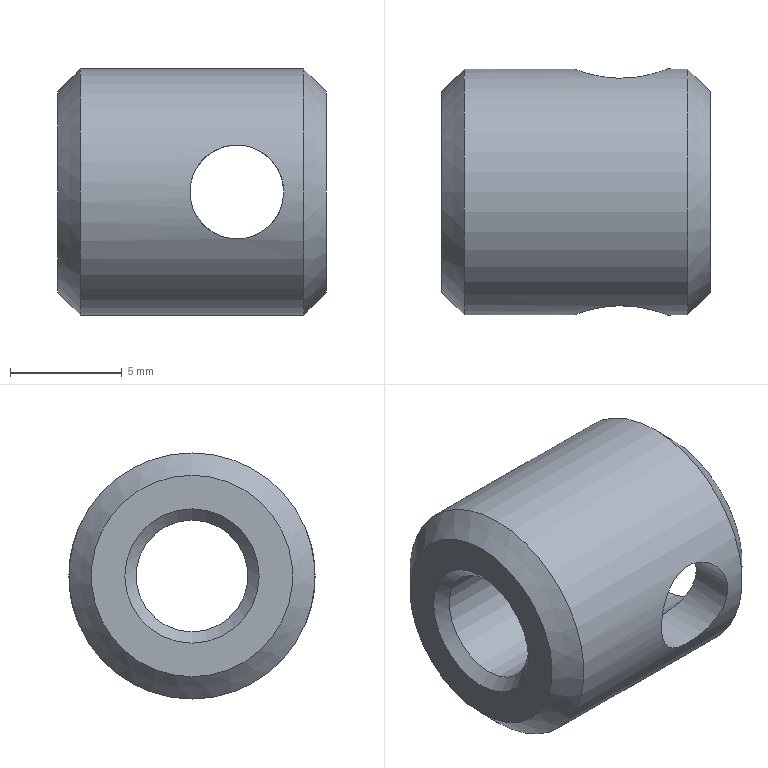Component | NX | 5_GAUGE_CLAMP_SLEEVE | 1 solid | 12 faces | volume 659 mm3 | cylinder 5 | cone 4 | plane 3 | commonest cylinder face diameters 4.2 x2 11 x1 7 x1 5 x1